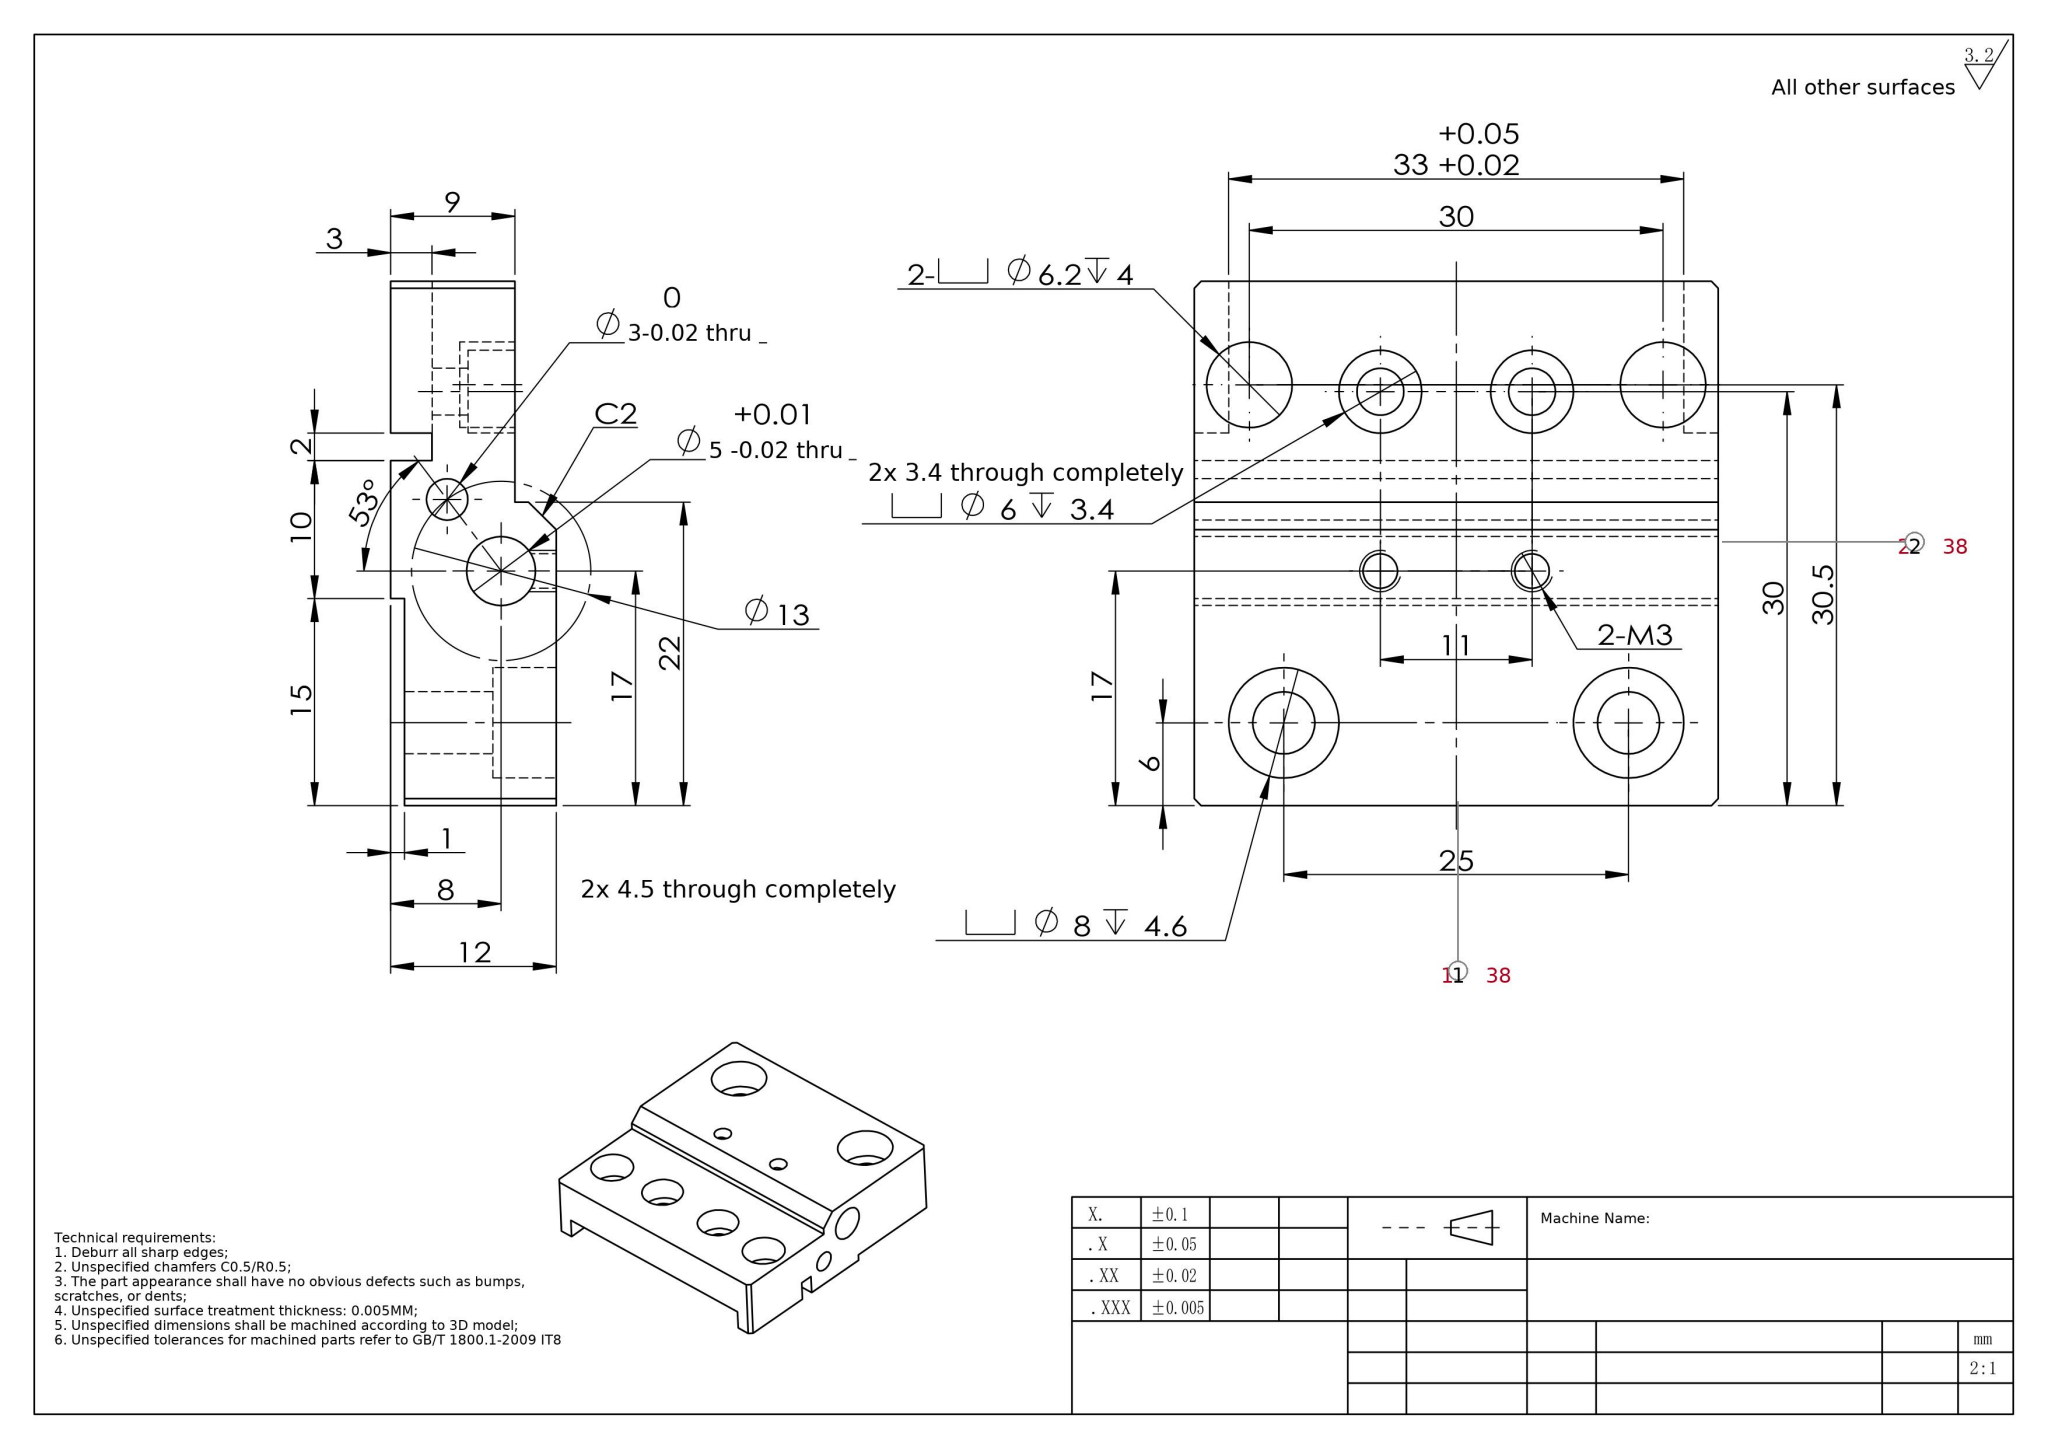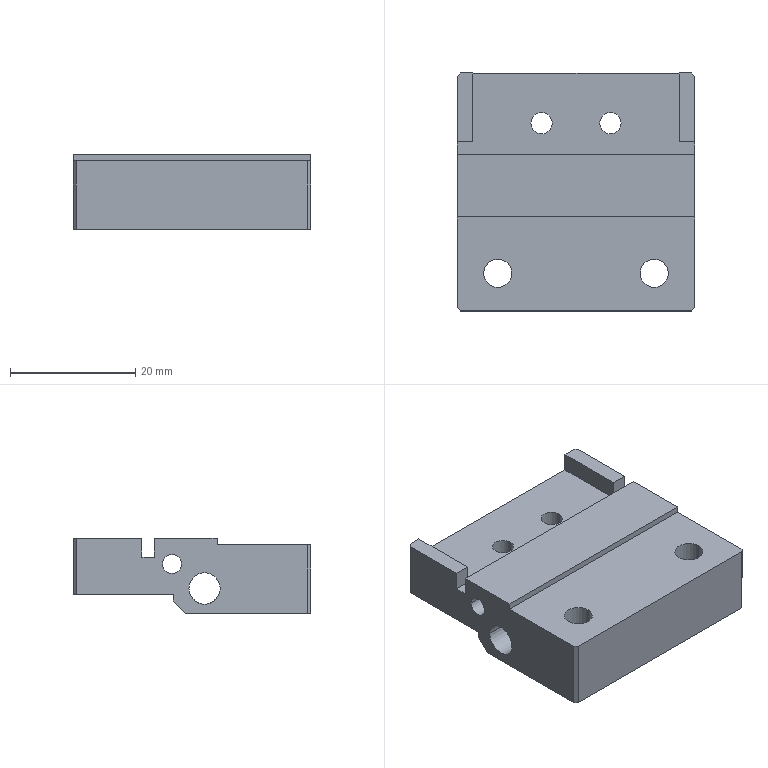Part | SolidWorks | mm | 1 solid | 57 faces | box 38 x 38 x 12 mm | volume 11359 mm3 | plane 29 | cylinder 28 | commonest cylinder face diameters 2.5 x4 8 x4 4.5 x4 6.2 x4 6 x4 3.4 x4 3 x2 5 x2
build123d program:
from build123d import *

# Parameters (mm, degrees)
SKETCH1_W                                            = 38
SKETCH1_H                                            = 38
BOSS_EXTRUDE1_DEPTH                                  = 6
SKETCH2_R                                            = 2.5
CUT_EXTRUDE1_DEPTH                                   = 43.907
SKETCH3_W                                            = 38
SKETCH3_H                                            = 16
CUT_EXTRUDE2_DEPTH                                   = 3
SKETCH4_R                                            = 1.5
CUT_EXTRUDE3_DEPTH                                   = 43.907
HOLE_SIZE_ACCORDING_TO_THE_TYPE_OF_HEXAG_D           = 3.4
HOLE_SIZE_ACCORDING_TO_THE_TYPE_OF_HEXAG_CBORE_D     = 6
HOLE_SIZE_ACCORDING_TO_THE_TYPE_OF_HEXAG_CBORE_DEPTH = 3.4
SKETCH11_R                                           = 3.1
CUT_EXTRUDE4_DEPTH                                   = 4
CUT_EXTRUDE5_DEPTH                                   = 3
SKETCH14_W                                           = 38
SKETCH14_H                                           = 15
CUT_EXTRUDE7_DEPTH                                   = 1
HOLE_SIZE_ACCORDING_TO_THE_TYPE_OF_H_2_D             = 4.5
HOLE_SIZE_ACCORDING_TO_THE_TYPE_OF_H_2_CBORE_D       = 8
HOLE_SIZE_ACCORDING_TO_THE_TYPE_OF_H_2_CBORE_DEPTH   = 4.6
M3_TAPPED_HOLE1_REACH                                = 31.428
M3_TAPPED_HOLE1_BORE_R                               = 1.25
CHAMFER1_SIZE                                        = 0.5
CHAMFER2_SIZE                                        = 2


with BuildPart() as part:
    # Sketch1 → Boss-Extrude1 (new, symmetric)
    with BuildSketch(Plane.XY):
        Rectangle(SKETCH1_W, SKETCH1_H)
    extrude(amount=BOSS_EXTRUDE1_DEPTH, both=True)

    # Sketch2 → Cut-Extrude1 (cut, through all)
    with BuildSketch(Plane.ZY.offset(19)):
        with Locations(Location((-2, -2, 0), (0, 0, 270))):
            Circle(SKETCH2_R)
    extrude(amount=-CUT_EXTRUDE1_DEPTH, mode=Mode.SUBTRACT)

    # Sketch3 → Cut-Extrude2 (cut)
    with BuildSketch(Plane(origin=(0, 0, -6), x_dir=(-1, 0, 0), z_dir=(0, 0, -1))):
        with Locations((0, 11)):
            Rectangle(SKETCH3_W, SKETCH3_H)
    extrude(amount=-CUT_EXTRUDE2_DEPTH, mode=Mode.SUBTRACT)

    # Sketch4 → Cut-Extrude3 (cut, through all)
    with BuildSketch(Plane.ZY.offset(19)):
        with Locations(Location((1.912, 3.191, 0), (0, 0, 270))):
            Circle(SKETCH4_R)
    extrude(amount=-CUT_EXTRUDE3_DEPTH, mode=Mode.SUBTRACT)

    # Hole Size according to the type of hexag (through all)
    with Locations(Plane(origin=(0, 0, -3), x_dir=(-1, 0, 0), z_dir=(0, 0, -1))):
        with Locations((-5.5, 11), (5.5, 11)):
            CounterBoreHole(HOLE_SIZE_ACCORDING_TO_THE_TYPE_OF_HEXAG_D / 2, HOLE_SIZE_ACCORDING_TO_THE_TYPE_OF_HEXAG_CBORE_D / 2, HOLE_SIZE_ACCORDING_TO_THE_TYPE_OF_HEXAG_CBORE_DEPTH)

    # Sketch11 → Cut-Extrude4 (cut)
    with BuildSketch(Plane(origin=(0, 0, -3), x_dir=(-1, 0, 0), z_dir=(0, 0, -1))):
        with Locations((-15, 11.5)):
            Circle(SKETCH11_R)
        with Locations((15, 11.5)):
            Circle(SKETCH11_R)
    extrude(amount=-CUT_EXTRUDE4_DEPTH, mode=Mode.SUBTRACT)

    # Sketch12 → Cut-Extrude5 (cut)
    with BuildSketch(Plane.XY.offset(6)):
        Polygon((16.5, 19), (-16.5, 19), (-16.5, 8), (-19, 8), (-19, 6), (19, 6), (19, 8), (16.5, 8), align=None)
    extrude(amount=-CUT_EXTRUDE5_DEPTH, mode=Mode.SUBTRACT)

    # Sketch14 → Cut-Extrude7 (cut)
    with BuildSketch(Plane.XY.offset(6)):
        with Locations((0, -11.5)):
            Rectangle(SKETCH14_W, SKETCH14_H)
    extrude(amount=-CUT_EXTRUDE7_DEPTH, mode=Mode.SUBTRACT)

    # Hole Size according to the type of h 2 (through all)
    with Locations(Plane(origin=(0, 0, -6), x_dir=(-1, 0, 0), z_dir=(0, 0, -1))):
        with Locations((-12.5, -13), (12.5, -13)):
            CounterBoreHole(HOLE_SIZE_ACCORDING_TO_THE_TYPE_OF_H_2_D / 2, HOLE_SIZE_ACCORDING_TO_THE_TYPE_OF_H_2_CBORE_D / 2, HOLE_SIZE_ACCORDING_TO_THE_TYPE_OF_H_2_CBORE_DEPTH)

    # M3 Tapped Hole1 bore → M3 Tapped Hole1 (cut, up to next)
    with BuildSketch(Plane(origin=(0, 0, -6), x_dir=(-1, 0, 0), z_dir=(0, 0, -1)), mode=Mode.PRIVATE) as m3_tapped_hole1_sk1:
        with Locations((5.5, -2)):
            Circle(M3_TAPPED_HOLE1_BORE_R)
    m3_tapped_hole1_tool1 = extrude(m3_tapped_hole1_sk1.sketch, amount=-M3_TAPPED_HOLE1_REACH, mode=Mode.PRIVATE) & part.part
    # M3 Tapped Hole1 bore → M3 Tapped Hole1 (cut, up to next)
    with BuildSketch(Plane(origin=(0, 0, -6), x_dir=(-1, 0, 0), z_dir=(0, 0, -1)), mode=Mode.PRIVATE) as m3_tapped_hole1_sk2:
        with Locations((-5.5, -2)):
            Circle(M3_TAPPED_HOLE1_BORE_R)
    m3_tapped_hole1_tool2 = extrude(m3_tapped_hole1_sk2.sketch, amount=-M3_TAPPED_HOLE1_REACH, mode=Mode.PRIVATE) & part.part
    add(m3_tapped_hole1_tool1.solids().sort_by_distance((-5.5, -2, -6))[0], mode=Mode.SUBTRACT)
    add(m3_tapped_hole1_tool2.solids().sort_by_distance((5.5, -2, -6))[0], mode=Mode.SUBTRACT)

    # Chamfer1
    chamfer1_edges = [part.edges().sort_by_distance(p)[0] for p in [
        (-19, 19, 1.5),
        (19, 19, 1.5),
        (19, -19, -0.5),
        (-19, -19, -0.5),
    ]]
    chamfer(chamfer1_edges, length=CHAMFER1_SIZE)

    # Chamfer2
    chamfer2_edges = [part.edges().sort_by_distance(p)[0] for p in [
        (0, 3, -6),
    ]]
    chamfer(chamfer2_edges, length=CHAMFER2_SIZE)


solid = part.part